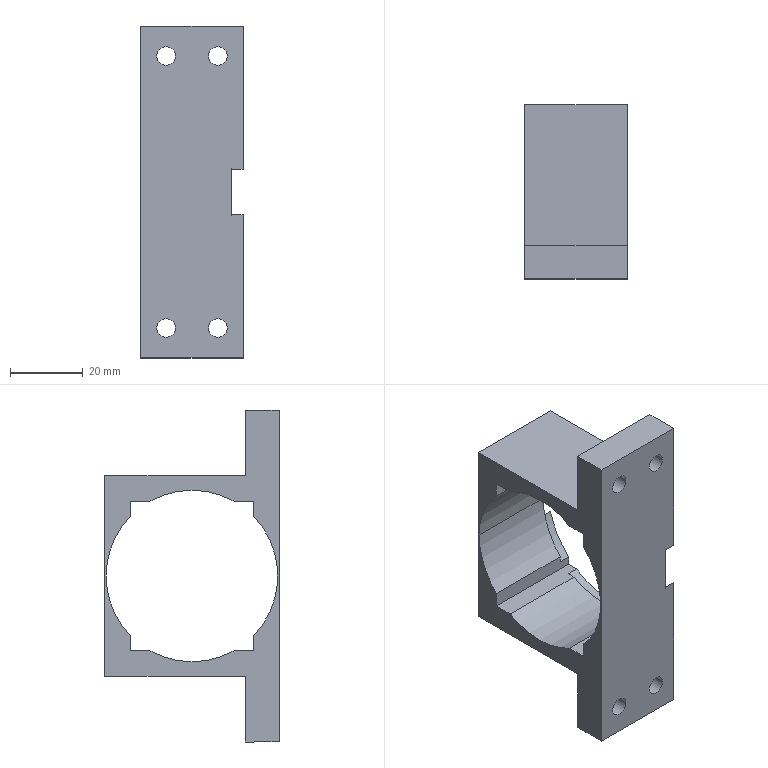Component | SolidWorks | EndCap-2 | 1 solid | 42 faces | volume 31961 mm3 | plane 23 | cylinder 19 | commonest cylinder face diameters 5.084 x8 49.4 x6 47.03 x5